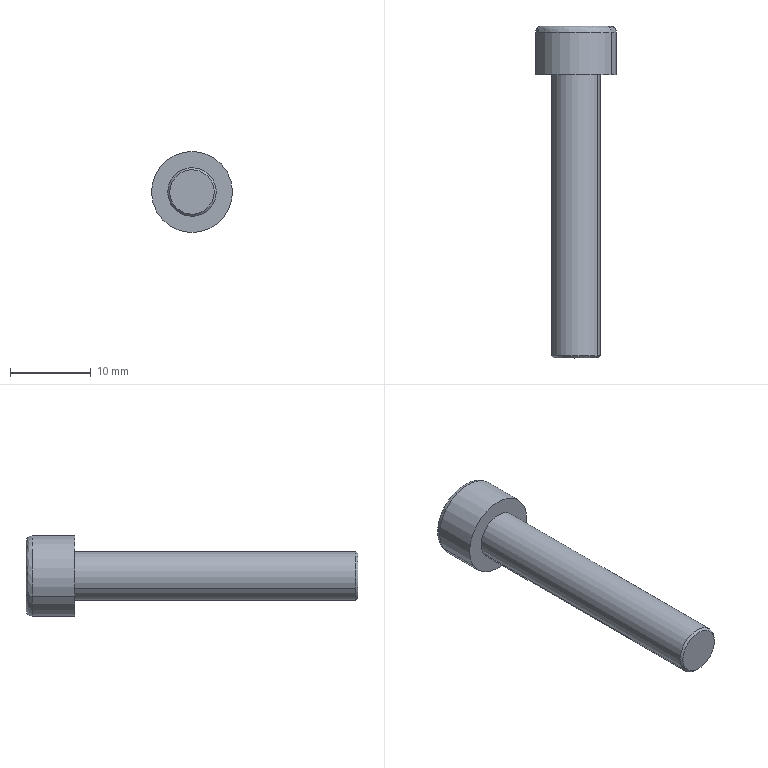Component | SolidWorks | ClampingAssembly-1_M6X35-N-1 | 1 solid | 25 faces | box 10 x 41 x 10 mm | volume 1382 mm3 | plane 15 | cylinder 4 | cone 4 | spline 2 | commonest cylinder face diameters 6 x2 10 x2 | material Standard Part
STEP:
#1=COLOUR_RGB('',0.7922,0.8196,0.9333);
#2=FILL_AREA_STYLE_COLOUR('',#1);
#3=FILL_AREA_STYLE('',(#2));
#4=SURFACE_STYLE_FILL_AREA(#3);
#5=SURFACE_SIDE_STYLE('',(#4));
#6=SURFACE_STYLE_USAGE(.BOTH.,#5);
#7=PRESENTATION_STYLE_ASSIGNMENT((#6));
#8=CARTESIAN_POINT('',(-0.1662,5.051,-1.732));
#9=VERTEX_POINT('',#8);
#10=CARTESIAN_POINT('',(-0.5071,5.051,-1.929));
#11=VERTEX_POINT('',#10);
#12=CARTESIAN_POINT('',(-0.3366,5.051,-1.831));
#13=DIRECTION('',(-0.,-1.,0.));
#14=DIRECTION('',(0.866,0.,0.5));
#15=AXIS2_PLACEMENT_3D('',#12,#13,#14);
#16=CIRCLE('',#15,0.1969);
#17=EDGE_CURVE('',#9,#11,#16,.T.);
#18=ORIENTED_EDGE('',*,*,#17,.F.);
#19=CARTESIAN_POINT('',(-0.1917,5.08,-1.747));
#20=VERTEX_POINT('',#19);
#21=CARTESIAN_POINT('',(-0.1917,5.051,-1.747));
#22=DIRECTION('',(-0.5,0.,0.866));
#23=DIRECTION('',(0.866,0.,0.5));
#24=AXIS2_PLACEMENT_3D('',#21,#22,#23);
#25=CIRCLE('',#24,0.02953);
#26=EDGE_CURVE('',#9,#20,#25,.T.);
#27=ORIENTED_EDGE('',*,*,#26,.T.);
#28=CARTESIAN_POINT('',(-0.4816,5.08,-1.914));
#29=VERTEX_POINT('',#28);
#30=CARTESIAN_POINT('',(-0.1917,5.08,-1.747));
#31=CARTESIAN_POINT('',(-0.3591,5.08,-1.457));
#32=CARTESIAN_POINT('',(-0.6489,5.08,-1.625));
#33=CARTESIAN_POINT('',(-0.4816,5.08,-1.914));
#34=(BOUNDED_CURVE()B_SPLINE_CURVE(3,(#30,#31,#32,#33),.UNSPECIFIED.,.F.,.F.)B_SPLINE_CURVE_WITH_KNOTS((4,4),(0.,1.),.UNSPECIFIED.)CURVE()GEOMETRIC_REPRESENTATION_ITEM()RATIONAL_B_SPLINE_CURVE((1.,0.3333,0.3333,1.))REPRESENTATION_ITEM(''));
#35=EDGE_CURVE('',#20,#29,#34,.T.);
#36=ORIENTED_EDGE('',*,*,#35,.T.);
#37=CARTESIAN_POINT('',(-0.4816,5.051,-1.914));
#38=DIRECTION('',(0.5,-0.,-0.866));
#39=DIRECTION('',(-0.866,0.,-0.5));
#40=AXIS2_PLACEMENT_3D('',#37,#38,#39);
#41=CIRCLE('',#40,0.02953);
#42=EDGE_CURVE('',#11,#29,#41,.T.);
#43=ORIENTED_EDGE('',*,*,#42,.F.);
#44=EDGE_LOOP('',(#18,#27,#36,#43));
#45=FACE_OUTER_BOUND('',#44,.T.);
#46=CARTESIAN_POINT('',(-0.1662,5.051,-1.732));
#47=CARTESIAN_POINT('',(-0.363,5.051,-1.391));
#48=CARTESIAN_POINT('',(-0.704,5.051,-1.588));
#49=CARTESIAN_POINT('',(-0.5071,5.051,-1.929));
#50=CARTESIAN_POINT('',(-0.1662,5.068,-1.732));
#51=CARTESIAN_POINT('',(-0.363,5.068,-1.391));
#52=CARTESIAN_POINT('',(-0.704,5.068,-1.588));
#53=CARTESIAN_POINT('',(-0.5071,5.068,-1.929));
#54=CARTESIAN_POINT('',(-0.1768,5.08,-1.738));
#55=CARTESIAN_POINT('',(-0.3614,5.08,-1.419));
#56=CARTESIAN_POINT('',(-0.6811,5.08,-1.603));
#57=CARTESIAN_POINT('',(-0.4965,5.08,-1.923));
#58=CARTESIAN_POINT('',(-0.1917,5.08,-1.747));
#59=CARTESIAN_POINT('',(-0.3591,5.08,-1.457));
#60=CARTESIAN_POINT('',(-0.6489,5.08,-1.625));
#61=CARTESIAN_POINT('',(-0.4816,5.08,-1.914));
#62=(BOUNDED_SURFACE()B_SPLINE_SURFACE(3,3,((#46,#47,#48,#49),(#50,#51,#52,#53),(#54,#55,#56,#57),(#58,#59,#60,#61)),.UNSPECIFIED.,.F.,.F.,.T.)B_SPLINE_SURFACE_WITH_KNOTS((4,4),(4,4),(0.,1.),(0.,1.),.UNSPECIFIED.)GEOMETRIC_REPRESENTATION_ITEM()RATIONAL_B_SPLINE_SURFACE(((1.,0.3333,0.3333,1.),(0.8047,0.2682,0.2682,0.8047),(0.8047,0.2682,0.2682,0.8047),(1.,0.3333,0.3333,1.)))REPRESENTATION_ITEM('')SURFACE());
#63=ADVANCED_FACE('',(#45),#62,.T.);
#64=CARTESIAN_POINT('',(-0.2344,3.476,-1.772));
#65=VERTEX_POINT('',#64);
#66=CARTESIAN_POINT('',(-0.4389,3.476,-1.89));
#67=VERTEX_POINT('',#66);
#68=CARTESIAN_POINT('',(-0.3366,3.476,-1.831));
#69=DIRECTION('',(0.,1.,-0.));
#70=DIRECTION('',(0.866,0.,0.5));
#71=AXIS2_PLACEMENT_3D('',#68,#69,#70);
#72=CIRCLE('',#71,0.1181);
#73=EDGE_CURVE('',#65,#67,#72,.T.);
#74=ORIENTED_EDGE('',*,*,#73,.T.);
#75=CARTESIAN_POINT('',(-0.4389,4.844,-1.89));
#76=VERTEX_POINT('',#75);
#77=CARTESIAN_POINT('',(-0.4389,3.466,-1.89));
#78=DIRECTION('',(0.,1.,-0.));
#79=VECTOR('',#78,39.37);
#80=LINE('',#77,#79);
#81=EDGE_CURVE('',#67,#76,#80,.T.);
#82=ORIENTED_EDGE('',*,*,#81,.T.);
#83=CARTESIAN_POINT('',(-0.2344,4.844,-1.772));
#84=VERTEX_POINT('',#83);
#85=CARTESIAN_POINT('',(-0.3366,4.844,-1.831));
#86=DIRECTION('',(-0.,-1.,0.));
#87=DIRECTION('',(0.866,0.,0.5));
#88=AXIS2_PLACEMENT_3D('',#85,#86,#87);
#89=CIRCLE('',#88,0.1181);
#90=EDGE_CURVE('',#76,#84,#89,.T.);
#91=ORIENTED_EDGE('',*,*,#90,.T.);
#92=CARTESIAN_POINT('',(-0.2344,3.466,-1.772));
#93=DIRECTION('',(0.,1.,-0.));
#94=VECTOR('',#93,39.37);
#95=LINE('',#92,#94);
#96=EDGE_CURVE('',#65,#84,#95,.T.);
#97=ORIENTED_EDGE('',*,*,#96,.F.);
#98=EDGE_LOOP('',(#74,#82,#91,#97));
#99=FACE_OUTER_BOUND('',#98,.T.);
#100=CARTESIAN_POINT('',(-0.3366,3.466,-1.831));
#101=DIRECTION('',(0.,1.,-0.));
#102=DIRECTION('',(0.866,0.,0.5));
#103=AXIS2_PLACEMENT_3D('',#100,#101,#102);
#104=CYLINDRICAL_SURFACE('',#103,0.1181);
#105=ADVANCED_FACE('',(#99),#104,.T.);
#106=CARTESIAN_POINT('',(-0.2429,3.466,-1.777));
#107=VERTEX_POINT('',#106);
#108=CARTESIAN_POINT('',(-0.4304,3.466,-1.885));
#109=VERTEX_POINT('',#108);
#110=CARTESIAN_POINT('',(-0.3366,3.466,-1.831));
#111=DIRECTION('',(0.,1.,-0.));
#112=DIRECTION('',(0.866,0.,0.5));
#113=AXIS2_PLACEMENT_3D('',#110,#111,#112);
#114=CIRCLE('',#113,0.1083);
#115=EDGE_CURVE('',#107,#109,#114,.T.);
#116=ORIENTED_EDGE('',*,*,#115,.T.);
#117=CARTESIAN_POINT('',(-0.4389,3.476,-1.89));
#118=DIRECTION('',(-0.6124,0.7071,-0.3536));
#119=VECTOR('',#118,39.37);
#120=LINE('',#117,#119);
#121=EDGE_CURVE('',#109,#67,#120,.T.);
#122=ORIENTED_EDGE('',*,*,#121,.T.);
#123=ORIENTED_EDGE('',*,*,#73,.F.);
#124=CARTESIAN_POINT('',(-0.2344,3.476,-1.772));
#125=DIRECTION('',(0.6124,0.7071,0.3536));
#126=VECTOR('',#125,39.37);
#127=LINE('',#124,#126);
#128=EDGE_CURVE('',#107,#65,#127,.T.);
#129=ORIENTED_EDGE('',*,*,#128,.F.);
#130=EDGE_LOOP('',(#116,#122,#123,#129));
#131=FACE_OUTER_BOUND('',#130,.T.);
#132=CARTESIAN_POINT('',(-0.3366,3.476,-1.831));
#133=DIRECTION('',(0.,1.,-0.));
#134=DIRECTION('',(0.866,0.,0.5));
#135=AXIS2_PLACEMENT_3D('',#132,#133,#134);
#136=CONICAL_SURFACE('',#135,0.1181,0.7854);
#137=ADVANCED_FACE('',(#131),#136,.T.);
#138=CARTESIAN_POINT('',(-0.5071,4.844,-1.929));
#139=VERTEX_POINT('',#138);
#140=CARTESIAN_POINT('',(-0.1662,4.844,-1.732));
#141=VERTEX_POINT('',#140);
#142=CARTESIAN_POINT('',(-0.3366,4.844,-1.831));
#143=DIRECTION('',(-0.,-1.,0.));
#144=DIRECTION('',(0.866,0.,0.5));
#145=AXIS2_PLACEMENT_3D('',#142,#143,#144);
#146=CIRCLE('',#145,0.1969);
#147=EDGE_CURVE('',#139,#141,#146,.T.);
#148=ORIENTED_EDGE('',*,*,#147,.F.);
#149=CARTESIAN_POINT('',(-0.5071,4.844,-1.929));
#150=DIRECTION('',(0.,1.,-0.));
#151=VECTOR('',#150,39.37);
#152=LINE('',#149,#151);
#153=EDGE_CURVE('',#139,#11,#152,.T.);
#154=ORIENTED_EDGE('',*,*,#153,.T.);
#155=CARTESIAN_POINT('',(-0.3366,5.051,-1.831));
#156=DIRECTION('',(-0.,-1.,0.));
#157=DIRECTION('',(0.866,0.,0.5));
#158=AXIS2_PLACEMENT_3D('',#155,#156,#157);
#159=CIRCLE('',#158,0.1969);
#160=EDGE_CURVE('',#11,#9,#159,.T.);
#161=ORIENTED_EDGE('',*,*,#160,.T.);
#162=CARTESIAN_POINT('',(-0.1662,4.844,-1.732));
#163=DIRECTION('',(0.,1.,-0.));
#164=VECTOR('',#163,39.37);
#165=LINE('',#162,#164);
#166=EDGE_CURVE('',#141,#9,#165,.T.);
#167=ORIENTED_EDGE('',*,*,#166,.F.);
#168=EDGE_LOOP('',(#148,#154,#161,#167));
#169=FACE_OUTER_BOUND('',#168,.T.);
#170=CARTESIAN_POINT('',(-0.3366,4.844,-1.831));
#171=DIRECTION('',(0.,1.,-0.));
#172=DIRECTION('',(0.866,0.,0.5));
#173=AXIS2_PLACEMENT_3D('',#170,#171,#172);
#174=CYLINDRICAL_SURFACE('',#173,0.1969);
#175=ADVANCED_FACE('',(#169),#174,.T.);
#176=CARTESIAN_POINT('',(-0.3366,4.905,-1.831));
#177=VERTEX_POINT('',#176);
#178=CARTESIAN_POINT('',(-0.2514,4.962,-1.781));
#179=VERTEX_POINT('',#178);
#180=CARTESIAN_POINT('',(-0.2514,4.962,-1.781));
#181=DIRECTION('',(0.75,0.5,0.433));
#182=VECTOR('',#181,39.37);
#183=LINE('',#180,#182);
#184=EDGE_CURVE('',#177,#179,#183,.T.);
#185=ORIENTED_EDGE('',*,*,#184,.F.);
#186=CARTESIAN_POINT('',(-0.4219,4.962,-1.88));
#187=VERTEX_POINT('',#186);
#188=CARTESIAN_POINT('',(-0.4219,4.962,-1.88));
#189=DIRECTION('',(-0.75,0.5,-0.433));
#190=VECTOR('',#189,39.37);
#191=LINE('',#188,#190);
#192=EDGE_CURVE('',#177,#187,#191,.T.);
#193=ORIENTED_EDGE('',*,*,#192,.T.);
#194=CARTESIAN_POINT('',(-0.4351,4.962,-1.831));
#195=VERTEX_POINT('',#194);
#196=CARTESIAN_POINT('',(-0.3366,4.962,-1.831));
#197=DIRECTION('',(-0.,-1.,0.));
#198=DIRECTION('',(0.866,0.,0.5));
#199=AXIS2_PLACEMENT_3D('',#196,#197,#198);
#200=CIRCLE('',#199,0.09843);
#201=EDGE_CURVE('',#195,#187,#200,.T.);
#202=ORIENTED_EDGE('',*,*,#201,.F.);
#203=CARTESIAN_POINT('',(-0.3859,4.962,-1.745));
#204=VERTEX_POINT('',#203);
#205=CARTESIAN_POINT('',(-0.3366,4.962,-1.831));
#206=DIRECTION('',(-0.,-1.,0.));
#207=DIRECTION('',(0.866,0.,0.5));
#208=AXIS2_PLACEMENT_3D('',#205,#206,#207);
#209=CIRCLE('',#208,0.09843);
#210=EDGE_CURVE('',#204,#195,#209,.T.);
#211=ORIENTED_EDGE('',*,*,#210,.F.);
#212=CARTESIAN_POINT('',(-0.2874,4.962,-1.745));
#213=VERTEX_POINT('',#212);
#214=CARTESIAN_POINT('',(-0.3366,4.962,-1.831));
#215=DIRECTION('',(-0.,-1.,0.));
#216=DIRECTION('',(0.866,0.,0.5));
#217=AXIS2_PLACEMENT_3D('',#214,#215,#216);
#218=CIRCLE('',#217,0.09843);
#219=EDGE_CURVE('',#213,#204,#218,.T.);
#220=ORIENTED_EDGE('',*,*,#219,.F.);
#221=CARTESIAN_POINT('',(-0.3366,4.962,-1.831));
#222=DIRECTION('',(-0.,-1.,0.));
#223=DIRECTION('',(0.866,0.,0.5));
#224=AXIS2_PLACEMENT_3D('',#221,#222,#223);
#225=CIRCLE('',#224,0.09843);
#226=EDGE_CURVE('',#179,#213,#225,.T.);
#227=ORIENTED_EDGE('',*,*,#226,.F.);
#228=EDGE_LOOP('',(#185,#193,#202,#211,#220,#227));
#229=FACE_OUTER_BOUND('',#228,.T.);
#230=CARTESIAN_POINT('',(-0.3366,4.962,-1.831));
#231=DIRECTION('',(0.,1.,-0.));
#232=DIRECTION('',(0.866,0.,0.5));
#233=AXIS2_PLACEMENT_3D('',#230,#231,#232);
#234=CONICAL_SURFACE('',#233,0.09843,1.047);
#235=ADVANCED_FACE('',(#229),#234,.F.);
#236=ORIENTED_EDGE('',*,*,#81,.F.);
#237=CARTESIAN_POINT('',(-0.3366,3.476,-1.831));
#238=DIRECTION('',(0.,1.,-0.));
#239=DIRECTION('',(0.866,0.,0.5));
#240=AXIS2_PLACEMENT_3D('',#237,#238,#239);
#241=CIRCLE('',#240,0.1181);
#242=EDGE_CURVE('',#67,#65,#241,.T.);
#243=ORIENTED_EDGE('',*,*,#242,.T.);
#244=ORIENTED_EDGE('',*,*,#96,.T.);
#245=CARTESIAN_POINT('',(-0.3366,4.844,-1.831));
#246=DIRECTION('',(-0.,-1.,0.));
#247=DIRECTION('',(0.866,0.,0.5));
#248=AXIS2_PLACEMENT_3D('',#245,#246,#247);
#249=CIRCLE('',#248,0.1181);
#250=EDGE_CURVE('',#84,#76,#249,.T.);
#251=ORIENTED_EDGE('',*,*,#250,.T.);
#252=EDGE_LOOP('',(#236,#243,#244,#251));
#253=FACE_OUTER_BOUND('',#252,.T.);
#254=CARTESIAN_POINT('',(-0.3366,3.466,-1.831));
#255=DIRECTION('',(0.,1.,-0.));
#256=DIRECTION('',(0.866,0.,0.5));
#257=AXIS2_PLACEMENT_3D('',#254,#255,#256);
#258=CYLINDRICAL_SURFACE('',#257,0.1181);
#259=ADVANCED_FACE('',(#253),#258,.T.);
#260=ORIENTED_EDGE('',*,*,#250,.F.);
#261=ORIENTED_EDGE('',*,*,#90,.F.);
#262=EDGE_LOOP('',(#260,#261));
#263=FACE_BOUND('',#262,.T.);
#264=CARTESIAN_POINT('',(-0.3366,4.844,-1.831));
#265=DIRECTION('',(-0.,-1.,0.));
#266=DIRECTION('',(0.866,0.,0.5));
#267=AXIS2_PLACEMENT_3D('',#264,#265,#266);
#268=CIRCLE('',#267,0.1969);
#269=EDGE_CURVE('',#141,#139,#268,.T.);
#270=ORIENTED_EDGE('',*,*,#269,.T.);
#271=ORIENTED_EDGE('',*,*,#147,.T.);
#272=EDGE_LOOP('',(#270,#271));
#273=FACE_OUTER_BOUND('',#272,.T.);
#274=CARTESIAN_POINT('',(-0.3366,4.844,-1.831));
#275=DIRECTION('',(-0.,-1.,0.));
#276=DIRECTION('',(-0.866,-0.,-0.5));
#277=AXIS2_PLACEMENT_3D('',#274,#275,#276);
#278=PLANE('',#277);
#279=ADVANCED_FACE('',(#263,#273),#278,.T.);
#280=ORIENTED_EDGE('',*,*,#121,.F.);
#281=CARTESIAN_POINT('',(-0.3366,3.466,-1.831));
#282=DIRECTION('',(0.,1.,-0.));
#283=DIRECTION('',(0.866,0.,0.5));
#284=AXIS2_PLACEMENT_3D('',#281,#282,#283);
#285=CIRCLE('',#284,0.1083);
#286=EDGE_CURVE('',#109,#107,#285,.T.);
#287=ORIENTED_EDGE('',*,*,#286,.T.);
#288=ORIENTED_EDGE('',*,*,#128,.T.);
#289=ORIENTED_EDGE('',*,*,#242,.F.);
#290=EDGE_LOOP('',(#280,#287,#288,#289));
#291=FACE_OUTER_BOUND('',#290,.T.);
#292=CARTESIAN_POINT('',(-0.3366,3.476,-1.831));
#293=DIRECTION('',(0.,1.,-0.));
#294=DIRECTION('',(0.866,0.,0.5));
#295=AXIS2_PLACEMENT_3D('',#292,#293,#294);
#296=CONICAL_SURFACE('',#295,0.1181,0.7854);
#297=ADVANCED_FACE('',(#291),#296,.T.);
#298=ORIENTED_EDGE('',*,*,#153,.F.);
#299=ORIENTED_EDGE('',*,*,#269,.F.);
#300=ORIENTED_EDGE('',*,*,#166,.T.);
#301=ORIENTED_EDGE('',*,*,#17,.T.);
#302=EDGE_LOOP('',(#298,#299,#300,#301));
#303=FACE_OUTER_BOUND('',#302,.T.);
#304=CARTESIAN_POINT('',(-0.3366,4.844,-1.831));
#305=DIRECTION('',(0.,1.,-0.));
#306=DIRECTION('',(0.866,0.,0.5));
#307=AXIS2_PLACEMENT_3D('',#304,#305,#306);
#308=CYLINDRICAL_SURFACE('',#307,0.1969);
#309=ADVANCED_FACE('',(#303),#308,.T.);
#310=ORIENTED_EDGE('',*,*,#115,.F.);
#311=ORIENTED_EDGE('',*,*,#286,.F.);
#312=EDGE_LOOP('',(#310,#311));
#313=FACE_OUTER_BOUND('',#312,.T.);
#314=CARTESIAN_POINT('',(-0.3366,3.466,-1.831));
#315=DIRECTION('',(-0.,-1.,0.));
#316=DIRECTION('',(-0.866,-0.,-0.5));
#317=AXIS2_PLACEMENT_3D('',#314,#315,#316);
#318=PLANE('',#317);
#319=ADVANCED_FACE('',(#313),#318,.T.);
#320=ORIENTED_EDGE('',*,*,#26,.F.);
#321=ORIENTED_EDGE('',*,*,#160,.F.);
#322=ORIENTED_EDGE('',*,*,#42,.T.);
#323=CARTESIAN_POINT('',(-0.4816,5.08,-1.914));
#324=CARTESIAN_POINT('',(-0.3142,5.08,-2.204));
#325=CARTESIAN_POINT('',(-0.02442,5.08,-2.037));
#326=CARTESIAN_POINT('',(-0.1917,5.08,-1.747));
#327=(BOUNDED_CURVE()B_SPLINE_CURVE(3,(#323,#324,#325,#326),.UNSPECIFIED.,.F.,.F.)B_SPLINE_CURVE_WITH_KNOTS((4,4),(0.,1.),.UNSPECIFIED.)CURVE()GEOMETRIC_REPRESENTATION_ITEM()RATIONAL_B_SPLINE_CURVE((1.,0.3333,0.3333,1.))REPRESENTATION_ITEM(''));
#328=EDGE_CURVE('',#29,#20,#327,.T.);
#329=ORIENTED_EDGE('',*,*,#328,.T.);
#330=EDGE_LOOP('',(#320,#321,#322,#329));
#331=FACE_OUTER_BOUND('',#330,.T.);
#332=CARTESIAN_POINT('',(-0.5071,5.051,-1.929));
#333=CARTESIAN_POINT('',(-0.3103,5.051,-2.27));
#334=CARTESIAN_POINT('',(0.03068,5.051,-2.073));
#335=CARTESIAN_POINT('',(-0.1662,5.051,-1.732));
#336=CARTESIAN_POINT('',(-0.5071,5.068,-1.929));
#337=CARTESIAN_POINT('',(-0.3103,5.068,-2.27));
#338=CARTESIAN_POINT('',(0.03068,5.068,-2.073));
#339=CARTESIAN_POINT('',(-0.1662,5.068,-1.732));
#340=CARTESIAN_POINT('',(-0.4965,5.08,-1.923));
#341=CARTESIAN_POINT('',(-0.3119,5.08,-2.243));
#342=CARTESIAN_POINT('',(0.007861,5.08,-2.058));
#343=CARTESIAN_POINT('',(-0.1768,5.08,-1.738));
#344=CARTESIAN_POINT('',(-0.4816,5.08,-1.914));
#345=CARTESIAN_POINT('',(-0.3142,5.08,-2.204));
#346=CARTESIAN_POINT('',(-0.02442,5.08,-2.037));
#347=CARTESIAN_POINT('',(-0.1917,5.08,-1.747));
#348=(BOUNDED_SURFACE()B_SPLINE_SURFACE(3,3,((#332,#333,#334,#335),(#336,#337,#338,#339),(#340,#341,#342,#343),(#344,#345,#346,#347)),.UNSPECIFIED.,.F.,.F.,.T.)B_SPLINE_SURFACE_WITH_KNOTS((4,4),(4,4),(0.,1.),(0.,1.),.UNSPECIFIED.)GEOMETRIC_REPRESENTATION_ITEM()RATIONAL_B_SPLINE_SURFACE(((1.,0.3333,0.3333,1.),(0.8047,0.2682,0.2682,0.8047),(0.8047,0.2682,0.2682,0.8047),(1.,0.3333,0.3333,1.)))REPRESENTATION_ITEM('')SURFACE());
#349=ADVANCED_FACE('',(#331),#348,.T.);
#350=CARTESIAN_POINT('',(-0.3366,5.08,-1.944));
#351=VERTEX_POINT('',#350);
#352=CARTESIAN_POINT('',(-0.4351,5.08,-1.888));
#353=VERTEX_POINT('',#352);
#354=CARTESIAN_POINT('',(-0.3366,5.08,-1.944));
#355=DIRECTION('',(-0.866,0.,0.5));
#356=VECTOR('',#355,39.37);
#357=LINE('',#354,#356);
#358=EDGE_CURVE('',#351,#353,#357,.T.);
#359=ORIENTED_EDGE('',*,*,#358,.F.);
#360=CARTESIAN_POINT('',(-0.2382,5.08,-1.888));
#361=VERTEX_POINT('',#360);
#362=CARTESIAN_POINT('',(-0.2874,5.08,-1.916));
#363=DIRECTION('',(-0.866,-0.,-0.5));
#364=VECTOR('',#363,39.37);
#365=LINE('',#362,#364);
#366=EDGE_CURVE('',#361,#351,#365,.T.);
#367=ORIENTED_EDGE('',*,*,#366,.F.);
#368=CARTESIAN_POINT('',(-0.2382,5.08,-1.774));
#369=VERTEX_POINT('',#368);
#370=CARTESIAN_POINT('',(-0.2382,5.08,-1.774));
#371=DIRECTION('',(-0.,-0.,-1.));
#372=VECTOR('',#371,39.37);
#373=LINE('',#370,#372);
#374=EDGE_CURVE('',#369,#361,#373,.T.);
#375=ORIENTED_EDGE('',*,*,#374,.F.);
#376=CARTESIAN_POINT('',(-0.3366,5.08,-1.717));
#377=VERTEX_POINT('',#376);
#378=CARTESIAN_POINT('',(-0.3366,5.08,-1.717));
#379=DIRECTION('',(0.866,-0.,-0.5));
#380=VECTOR('',#379,39.37);
#381=LINE('',#378,#380);
#382=EDGE_CURVE('',#377,#369,#381,.T.);
#383=ORIENTED_EDGE('',*,*,#382,.F.);
#384=CARTESIAN_POINT('',(-0.4351,5.08,-1.774));
#385=VERTEX_POINT('',#384);
#386=CARTESIAN_POINT('',(-0.3859,5.08,-1.745));
#387=DIRECTION('',(0.866,0.,0.5));
#388=VECTOR('',#387,39.37);
#389=LINE('',#386,#388);
#390=EDGE_CURVE('',#385,#377,#389,.T.);
#391=ORIENTED_EDGE('',*,*,#390,.F.);
#392=CARTESIAN_POINT('',(-0.4351,5.08,-1.888));
#393=DIRECTION('',(0.,0.,1.));
#394=VECTOR('',#393,39.37);
#395=LINE('',#392,#394);
#396=EDGE_CURVE('',#353,#385,#395,.T.);
#397=ORIENTED_EDGE('',*,*,#396,.F.);
#398=EDGE_LOOP('',(#359,#367,#375,#383,#391,#397));
#399=FACE_BOUND('',#398,.T.);
#400=ORIENTED_EDGE('',*,*,#328,.F.);
#401=ORIENTED_EDGE('',*,*,#35,.F.);
#402=EDGE_LOOP('',(#400,#401));
#403=FACE_OUTER_BOUND('',#402,.T.);
#404=CARTESIAN_POINT('',(-0.3366,5.08,-1.831));
#405=DIRECTION('',(-0.,-1.,0.));
#406=DIRECTION('',(-0.866,-0.,-0.5));
#407=AXIS2_PLACEMENT_3D('',#404,#405,#406);
#408=PLANE('',#407);
#409=ADVANCED_FACE('',(#399,#403),#408,.F.);
#410=CARTESIAN_POINT('',(-0.4351,4.962,-1.888));
#411=VERTEX_POINT('',#410);
#412=CARTESIAN_POINT('',(-0.4351,4.962,-1.774));
#413=DIRECTION('',(-0.,-0.,-1.));
#414=VECTOR('',#413,39.37);
#415=LINE('',#412,#414);
#416=EDGE_CURVE('',#195,#411,#415,.T.);
#417=ORIENTED_EDGE('',*,*,#416,.T.);
#418=CARTESIAN_POINT('',(-0.4351,4.962,-1.888));
#419=DIRECTION('',(0.,1.,-0.));
#420=VECTOR('',#419,39.37);
#421=LINE('',#418,#420);
#422=EDGE_CURVE('',#411,#353,#421,.T.);
#423=ORIENTED_EDGE('',*,*,#422,.T.);
#424=ORIENTED_EDGE('',*,*,#396,.T.);
#425=CARTESIAN_POINT('',(-0.4351,4.962,-1.774));
#426=VERTEX_POINT('',#425);
#427=CARTESIAN_POINT('',(-0.4351,4.962,-1.774));
#428=DIRECTION('',(-0.,-1.,0.));
#429=VECTOR('',#428,39.37);
#430=LINE('',#427,#429);
#431=EDGE_CURVE('',#385,#426,#430,.T.);
#432=ORIENTED_EDGE('',*,*,#431,.T.);
#433=CARTESIAN_POINT('',(-0.4351,4.962,-1.831));
#434=DIRECTION('',(0.,0.,1.));
#435=VECTOR('',#434,39.37);
#436=LINE('',#433,#435);
#437=EDGE_CURVE('',#195,#426,#436,.T.);
#438=ORIENTED_EDGE('',*,*,#437,.F.);
#439=EDGE_LOOP('',(#417,#423,#424,#432,#438));
#440=FACE_OUTER_BOUND('',#439,.T.);
#441=CARTESIAN_POINT('',(-0.4351,4.962,-1.774));
#442=DIRECTION('',(1.,-0.,-0.));
#443=DIRECTION('',(0.,0.,1.));
#444=AXIS2_PLACEMENT_3D('',#441,#442,#443);
#445=PLANE('',#444);
#446=ADVANCED_FACE('',(#440),#445,.T.);
#447=CARTESIAN_POINT('',(-0.3366,4.962,-1.944));
#448=VERTEX_POINT('',#447);
#449=CARTESIAN_POINT('',(-0.3859,4.962,-1.916));
#450=VERTEX_POINT('',#449);
#451=CARTESIAN_POINT('',(-0.3366,4.962,-1.944));
#452=DIRECTION('',(-0.866,0.,0.5));
#453=VECTOR('',#452,39.37);
#454=LINE('',#451,#453);
#455=EDGE_CURVE('',#448,#450,#454,.T.);
#456=ORIENTED_EDGE('',*,*,#455,.F.);
#457=CARTESIAN_POINT('',(-0.3366,4.962,-1.944));
#458=DIRECTION('',(0.,1.,-0.));
#459=VECTOR('',#458,39.37);
#460=LINE('',#457,#459);
#461=EDGE_CURVE('',#448,#351,#460,.T.);
#462=ORIENTED_EDGE('',*,*,#461,.T.);
#463=ORIENTED_EDGE('',*,*,#358,.T.);
#464=ORIENTED_EDGE('',*,*,#422,.F.);
#465=CARTESIAN_POINT('',(-0.4351,4.962,-1.888));
#466=DIRECTION('',(0.866,-0.,-0.5));
#467=VECTOR('',#466,39.37);
#468=LINE('',#465,#467);
#469=EDGE_CURVE('',#411,#450,#468,.T.);
#470=ORIENTED_EDGE('',*,*,#469,.T.);
#471=EDGE_LOOP('',(#456,#462,#463,#464,#470));
#472=FACE_OUTER_BOUND('',#471,.T.);
#473=CARTESIAN_POINT('',(-0.4351,4.962,-1.888));
#474=DIRECTION('',(0.5,0.,0.866));
#475=DIRECTION('',(-0.866,0.,0.5));
#476=AXIS2_PLACEMENT_3D('',#473,#474,#475);
#477=PLANE('',#476);
#478=ADVANCED_FACE('',(#472),#477,.T.);
#479=CARTESIAN_POINT('',(-0.2382,4.962,-1.888));
#480=VERTEX_POINT('',#479);
#481=CARTESIAN_POINT('',(-0.2874,4.962,-1.916));
#482=VERTEX_POINT('',#481);
#483=CARTESIAN_POINT('',(-0.2874,4.962,-1.916));
#484=DIRECTION('',(-0.866,-0.,-0.5));
#485=VECTOR('',#484,39.37);
#486=LINE('',#483,#485);
#487=EDGE_CURVE('',#480,#482,#486,.T.);
#488=ORIENTED_EDGE('',*,*,#487,.F.);
#489=CARTESIAN_POINT('',(-0.2382,4.962,-1.888));
#490=DIRECTION('',(0.,1.,-0.));
#491=VECTOR('',#490,39.37);
#492=LINE('',#489,#491);
#493=EDGE_CURVE('',#480,#361,#492,.T.);
#494=ORIENTED_EDGE('',*,*,#493,.T.);
#495=ORIENTED_EDGE('',*,*,#366,.T.);
#496=ORIENTED_EDGE('',*,*,#461,.F.);
#497=CARTESIAN_POINT('',(-0.2874,4.962,-1.916));
#498=DIRECTION('',(-0.866,-0.,-0.5));
#499=VECTOR('',#498,39.37);
#500=LINE('',#497,#499);
#501=EDGE_CURVE('',#482,#448,#500,.T.);
#502=ORIENTED_EDGE('',*,*,#501,.F.);
#503=EDGE_LOOP('',(#488,#494,#495,#496,#502));
#504=FACE_OUTER_BOUND('',#503,.T.);
#505=CARTESIAN_POINT('',(-0.3366,4.962,-1.944));
#506=DIRECTION('',(-0.5,0.,0.866));
#507=DIRECTION('',(-0.866,-0.,-0.5));
#508=AXIS2_PLACEMENT_3D('',#505,#506,#507);
#509=PLANE('',#508);
#510=ADVANCED_FACE('',(#504),#509,.T.);
#511=CARTESIAN_POINT('',(-0.2382,4.962,-1.831));
#512=VERTEX_POINT('',#511);
#513=CARTESIAN_POINT('',(-0.2382,4.962,-1.774));
#514=VERTEX_POINT('',#513);
#515=CARTESIAN_POINT('',(-0.2382,4.962,-1.888));
#516=DIRECTION('',(0.,0.,1.));
#517=VECTOR('',#516,39.37);
#518=LINE('',#515,#517);
#519=EDGE_CURVE('',#512,#514,#518,.T.);
#520=ORIENTED_EDGE('',*,*,#519,.T.);
#521=CARTESIAN_POINT('',(-0.2382,4.962,-1.774));
#522=DIRECTION('',(0.,1.,-0.));
#523=VECTOR('',#522,39.37);
#524=LINE('',#521,#523);
#525=EDGE_CURVE('',#514,#369,#524,.T.);
#526=ORIENTED_EDGE('',*,*,#525,.T.);
#527=ORIENTED_EDGE('',*,*,#374,.T.);
#528=ORIENTED_EDGE('',*,*,#493,.F.);
#529=CARTESIAN_POINT('',(-0.2382,4.962,-1.831));
#530=DIRECTION('',(0.,-0.,-1.));
#531=VECTOR('',#530,39.37);
#532=LINE('',#529,#531);
#533=EDGE_CURVE('',#512,#480,#532,.T.);
#534=ORIENTED_EDGE('',*,*,#533,.F.);
#535=EDGE_LOOP('',(#520,#526,#527,#528,#534));
#536=FACE_OUTER_BOUND('',#535,.T.);
#537=CARTESIAN_POINT('',(-0.2382,4.962,-1.888));
#538=DIRECTION('',(-1.,0.,0.));
#539=DIRECTION('',(-0.,-0.,-1.));
#540=AXIS2_PLACEMENT_3D('',#537,#538,#539);
#541=PLANE('',#540);
#542=ADVANCED_FACE('',(#536),#541,.T.);
#543=CARTESIAN_POINT('',(-0.3366,4.962,-1.717));
#544=VERTEX_POINT('',#543);
#545=CARTESIAN_POINT('',(-0.2382,4.962,-1.774));
#546=DIRECTION('',(-0.866,0.,0.5));
#547=VECTOR('',#546,39.37);
#548=LINE('',#545,#547);
#549=EDGE_CURVE('',#213,#544,#548,.T.);
#550=ORIENTED_EDGE('',*,*,#549,.T.);
#551=CARTESIAN_POINT('',(-0.3366,4.962,-1.717));
#552=DIRECTION('',(0.,1.,-0.));
#553=VECTOR('',#552,39.37);
#554=LINE('',#551,#553);
#555=EDGE_CURVE('',#544,#377,#554,.T.);
#556=ORIENTED_EDGE('',*,*,#555,.T.);
#557=ORIENTED_EDGE('',*,*,#382,.T.);
#558=ORIENTED_EDGE('',*,*,#525,.F.);
#559=CARTESIAN_POINT('',(-0.2382,4.962,-1.774));
#560=DIRECTION('',(-0.866,0.,0.5));
#561=VECTOR('',#560,39.37);
#562=LINE('',#559,#561);
#563=EDGE_CURVE('',#514,#213,#562,.T.);
#564=ORIENTED_EDGE('',*,*,#563,.T.);
#565=EDGE_LOOP('',(#550,#556,#557,#558,#564));
#566=FACE_OUTER_BOUND('',#565,.T.);
#567=CARTESIAN_POINT('',(-0.2382,4.962,-1.774));
#568=DIRECTION('',(-0.5,-0.,-0.866));
#569=DIRECTION('',(0.866,-0.,-0.5));
#570=AXIS2_PLACEMENT_3D('',#567,#568,#569);
#571=PLANE('',#570);
#572=ADVANCED_FACE('',(#566),#571,.T.);
#573=CARTESIAN_POINT('',(-0.3859,4.962,-1.745));
#574=DIRECTION('',(0.866,0.,0.5));
#575=VECTOR('',#574,39.37);
#576=LINE('',#573,#575);
#577=EDGE_CURVE('',#426,#204,#576,.T.);
#578=ORIENTED_EDGE('',*,*,#577,.F.);
#579=ORIENTED_EDGE('',*,*,#431,.F.);
#580=ORIENTED_EDGE('',*,*,#390,.T.);
#581=ORIENTED_EDGE('',*,*,#555,.F.);
#582=CARTESIAN_POINT('',(-0.3366,4.962,-1.717));
#583=DIRECTION('',(-0.866,-0.,-0.5));
#584=VECTOR('',#583,39.37);
#585=LINE('',#582,#584);
#586=EDGE_CURVE('',#544,#204,#585,.T.);
#587=ORIENTED_EDGE('',*,*,#586,.T.);
#588=EDGE_LOOP('',(#578,#579,#580,#581,#587));
#589=FACE_OUTER_BOUND('',#588,.T.);
#590=CARTESIAN_POINT('',(-0.3366,4.962,-1.717));
#591=DIRECTION('',(0.5,-0.,-0.866));
#592=DIRECTION('',(0.866,0.,0.5));
#593=AXIS2_PLACEMENT_3D('',#590,#591,#592);
#594=PLANE('',#593);
#595=ADVANCED_FACE('',(#589),#594,.T.);
#596=ORIENTED_EDGE('',*,*,#201,.T.);
#597=CARTESIAN_POINT('',(-0.3366,4.962,-1.831));
#598=DIRECTION('',(-0.,-1.,0.));
#599=DIRECTION('',(0.866,0.,0.5));
#600=AXIS2_PLACEMENT_3D('',#597,#598,#599);
#601=CIRCLE('',#600,0.09843);
#602=EDGE_CURVE('',#187,#450,#601,.T.);
#603=ORIENTED_EDGE('',*,*,#602,.T.);
#604=ORIENTED_EDGE('',*,*,#469,.F.);
#605=ORIENTED_EDGE('',*,*,#416,.F.);
#606=EDGE_LOOP('',(#596,#603,#604,#605));
#607=FACE_OUTER_BOUND('',#606,.T.);
#608=CARTESIAN_POINT('',(-0.4351,4.962,-1.66));
#609=DIRECTION('',(0.,1.,-0.));
#610=DIRECTION('',(0.866,0.,0.5));
#611=AXIS2_PLACEMENT_3D('',#608,#609,#610);
#612=PLANE('',#611);
#613=ADVANCED_FACE('',(#607),#612,.T.);
#614=CARTESIAN_POINT('',(-0.3366,4.962,-1.831));
#615=DIRECTION('',(-0.,-1.,0.));
#616=DIRECTION('',(0.866,0.,0.5));
#617=AXIS2_PLACEMENT_3D('',#614,#615,#616);
#618=CIRCLE('',#617,0.09843);
#619=EDGE_CURVE('',#512,#179,#618,.T.);
#620=ORIENTED_EDGE('',*,*,#619,.T.);
#621=ORIENTED_EDGE('',*,*,#226,.T.);
#622=ORIENTED_EDGE('',*,*,#563,.F.);
#623=ORIENTED_EDGE('',*,*,#519,.F.);
#624=EDGE_LOOP('',(#620,#621,#622,#623));
#625=FACE_OUTER_BOUND('',#624,.T.);
#626=CARTESIAN_POINT('',(-0.4351,4.962,-1.66));
#627=DIRECTION('',(0.,1.,-0.));
#628=DIRECTION('',(0.866,0.,0.5));
#629=AXIS2_PLACEMENT_3D('',#626,#627,#628);
#630=PLANE('',#629);
#631=ADVANCED_FACE('',(#625),#630,.T.);
#632=ORIENTED_EDGE('',*,*,#219,.T.);
#633=ORIENTED_EDGE('',*,*,#586,.F.);
#634=ORIENTED_EDGE('',*,*,#549,.F.);
#635=EDGE_LOOP('',(#632,#633,#634));
#636=FACE_OUTER_BOUND('',#635,.T.);
#637=CARTESIAN_POINT('',(-0.4351,4.962,-1.66));
#638=DIRECTION('',(0.,1.,-0.));
#639=DIRECTION('',(0.866,0.,0.5));
#640=AXIS2_PLACEMENT_3D('',#637,#638,#639);
#641=PLANE('',#640);
#642=ADVANCED_FACE('',(#636),#641,.T.);
#643=ORIENTED_EDGE('',*,*,#192,.F.);
#644=ORIENTED_EDGE('',*,*,#184,.T.);
#645=ORIENTED_EDGE('',*,*,#619,.F.);
#646=CARTESIAN_POINT('',(-0.3366,4.962,-1.831));
#647=DIRECTION('',(-0.,-1.,0.));
#648=DIRECTION('',(0.866,0.,0.5));
#649=AXIS2_PLACEMENT_3D('',#646,#647,#648);
#650=CIRCLE('',#649,0.09843);
#651=EDGE_CURVE('',#482,#512,#650,.T.);
#652=ORIENTED_EDGE('',*,*,#651,.F.);
#653=CARTESIAN_POINT('',(-0.3366,4.962,-1.831));
#654=DIRECTION('',(-0.,-1.,0.));
#655=DIRECTION('',(0.866,0.,0.5));
#656=AXIS2_PLACEMENT_3D('',#653,#654,#655);
#657=CIRCLE('',#656,0.09843);
#658=EDGE_CURVE('',#450,#482,#657,.T.);
#659=ORIENTED_EDGE('',*,*,#658,.F.);
#660=ORIENTED_EDGE('',*,*,#602,.F.);
#661=EDGE_LOOP('',(#643,#644,#645,#652,#659,#660));
#662=FACE_OUTER_BOUND('',#661,.T.);
#663=CARTESIAN_POINT('',(-0.3366,4.962,-1.831));
#664=DIRECTION('',(0.,1.,-0.));
#665=DIRECTION('',(0.866,0.,0.5));
#666=AXIS2_PLACEMENT_3D('',#663,#664,#665);
#667=CONICAL_SURFACE('',#666,0.09843,1.047);
#668=ADVANCED_FACE('',(#662),#667,.F.);
#669=ORIENTED_EDGE('',*,*,#210,.T.);
#670=ORIENTED_EDGE('',*,*,#437,.T.);
#671=ORIENTED_EDGE('',*,*,#577,.T.);
#672=EDGE_LOOP('',(#669,#670,#671));
#673=FACE_OUTER_BOUND('',#672,.T.);
#674=CARTESIAN_POINT('',(-0.4351,4.962,-1.66));
#675=DIRECTION('',(0.,1.,-0.));
#676=DIRECTION('',(0.866,0.,0.5));
#677=AXIS2_PLACEMENT_3D('',#674,#675,#676);
#678=PLANE('',#677);
#679=ADVANCED_FACE('',(#673),#678,.T.);
#680=ORIENTED_EDGE('',*,*,#651,.T.);
#681=ORIENTED_EDGE('',*,*,#533,.T.);
#682=ORIENTED_EDGE('',*,*,#487,.T.);
#683=EDGE_LOOP('',(#680,#681,#682));
#684=FACE_OUTER_BOUND('',#683,.T.);
#685=CARTESIAN_POINT('',(-0.4351,4.962,-1.66));
#686=DIRECTION('',(0.,1.,-0.));
#687=DIRECTION('',(0.866,0.,0.5));
#688=AXIS2_PLACEMENT_3D('',#685,#686,#687);
#689=PLANE('',#688);
#690=ADVANCED_FACE('',(#684),#689,.T.);
#691=ORIENTED_EDGE('',*,*,#658,.T.);
#692=ORIENTED_EDGE('',*,*,#501,.T.);
#693=ORIENTED_EDGE('',*,*,#455,.T.);
#694=EDGE_LOOP('',(#691,#692,#693));
#695=FACE_OUTER_BOUND('',#694,.T.);
#696=CARTESIAN_POINT('',(-0.4351,4.962,-1.66));
#697=DIRECTION('',(0.,1.,-0.));
#698=DIRECTION('',(0.866,0.,0.5));
#699=AXIS2_PLACEMENT_3D('',#696,#697,#698);
#700=PLANE('',#699);
#701=ADVANCED_FACE('',(#695),#700,.T.);
#702=CLOSED_SHELL('',(#63,#105,#137,#175,#235,#259,#279,#297,#309,#319,#349,#409,#446,#478,#510,#542,#572,#595,#613,#631,#642,#668,#679,#690,#701));
#703=MANIFOLD_SOLID_BREP('',#702);
#704=STYLED_ITEM('',(#7),#703);
#705=(LENGTH_UNIT()NAMED_UNIT(*)SI_UNIT($,.METRE.));
#706=LENGTH_MEASURE_WITH_UNIT(LENGTH_MEASURE(0.0254),#705);
#707=DIMENSIONAL_EXPONENTS(1.,0.,0.,0.,0.,0.,0.);
#708=(CONVERSION_BASED_UNIT('',#706)LENGTH_UNIT()NAMED_UNIT(#707));
#709=UNCERTAINTY_MEASURE_WITH_UNIT(LENGTH_MEASURE(0.00001),#708,'','');
#710=(NAMED_UNIT(*)PLANE_ANGLE_UNIT()SI_UNIT($,.RADIAN.));
#711=(NAMED_UNIT(*)SI_UNIT($,.STERADIAN.)SOLID_ANGLE_UNIT());
#712=(GEOMETRIC_REPRESENTATION_CONTEXT(3)GLOBAL_UNCERTAINTY_ASSIGNED_CONTEXT((#709))GLOBAL_UNIT_ASSIGNED_CONTEXT((#708,#710,#711))REPRESENTATION_CONTEXT('',''));
#713=MECHANICAL_DESIGN_GEOMETRIC_PRESENTATION_REPRESENTATION('',(#704),#712);
#714=PRESENTATION_LAYER_ASSIGNMENT('','',(#704));
#715=CARTESIAN_POINT('',(0.,0.,0.));
#716=DIRECTION('',(0.,0.,1.));
#717=DIRECTION('',(1.,0.,0.));
#718=AXIS2_PLACEMENT_3D('',#715,#716,#717);
#719=(LENGTH_UNIT()NAMED_UNIT(*)SI_UNIT($,.METRE.));
#720=LENGTH_MEASURE_WITH_UNIT(LENGTH_MEASURE(0.0254),#719);
#721=DIMENSIONAL_EXPONENTS(1.,0.,0.,0.,0.,0.,0.);
#722=(CONVERSION_BASED_UNIT('',#720)LENGTH_UNIT()NAMED_UNIT(#721));
#723=UNCERTAINTY_MEASURE_WITH_UNIT(LENGTH_MEASURE(0.00001),#722,'','');
#724=(NAMED_UNIT(*)PLANE_ANGLE_UNIT()SI_UNIT($,.RADIAN.));
#725=(NAMED_UNIT(*)SI_UNIT($,.STERADIAN.)SOLID_ANGLE_UNIT());
#726=(GEOMETRIC_REPRESENTATION_CONTEXT(3)GLOBAL_UNCERTAINTY_ASSIGNED_CONTEXT((#723))GLOBAL_UNIT_ASSIGNED_CONTEXT((#722,#724,#725))REPRESENTATION_CONTEXT('',''));
#727=ADVANCED_BREP_SHAPE_REPRESENTATION('',(#703,#718),#726);